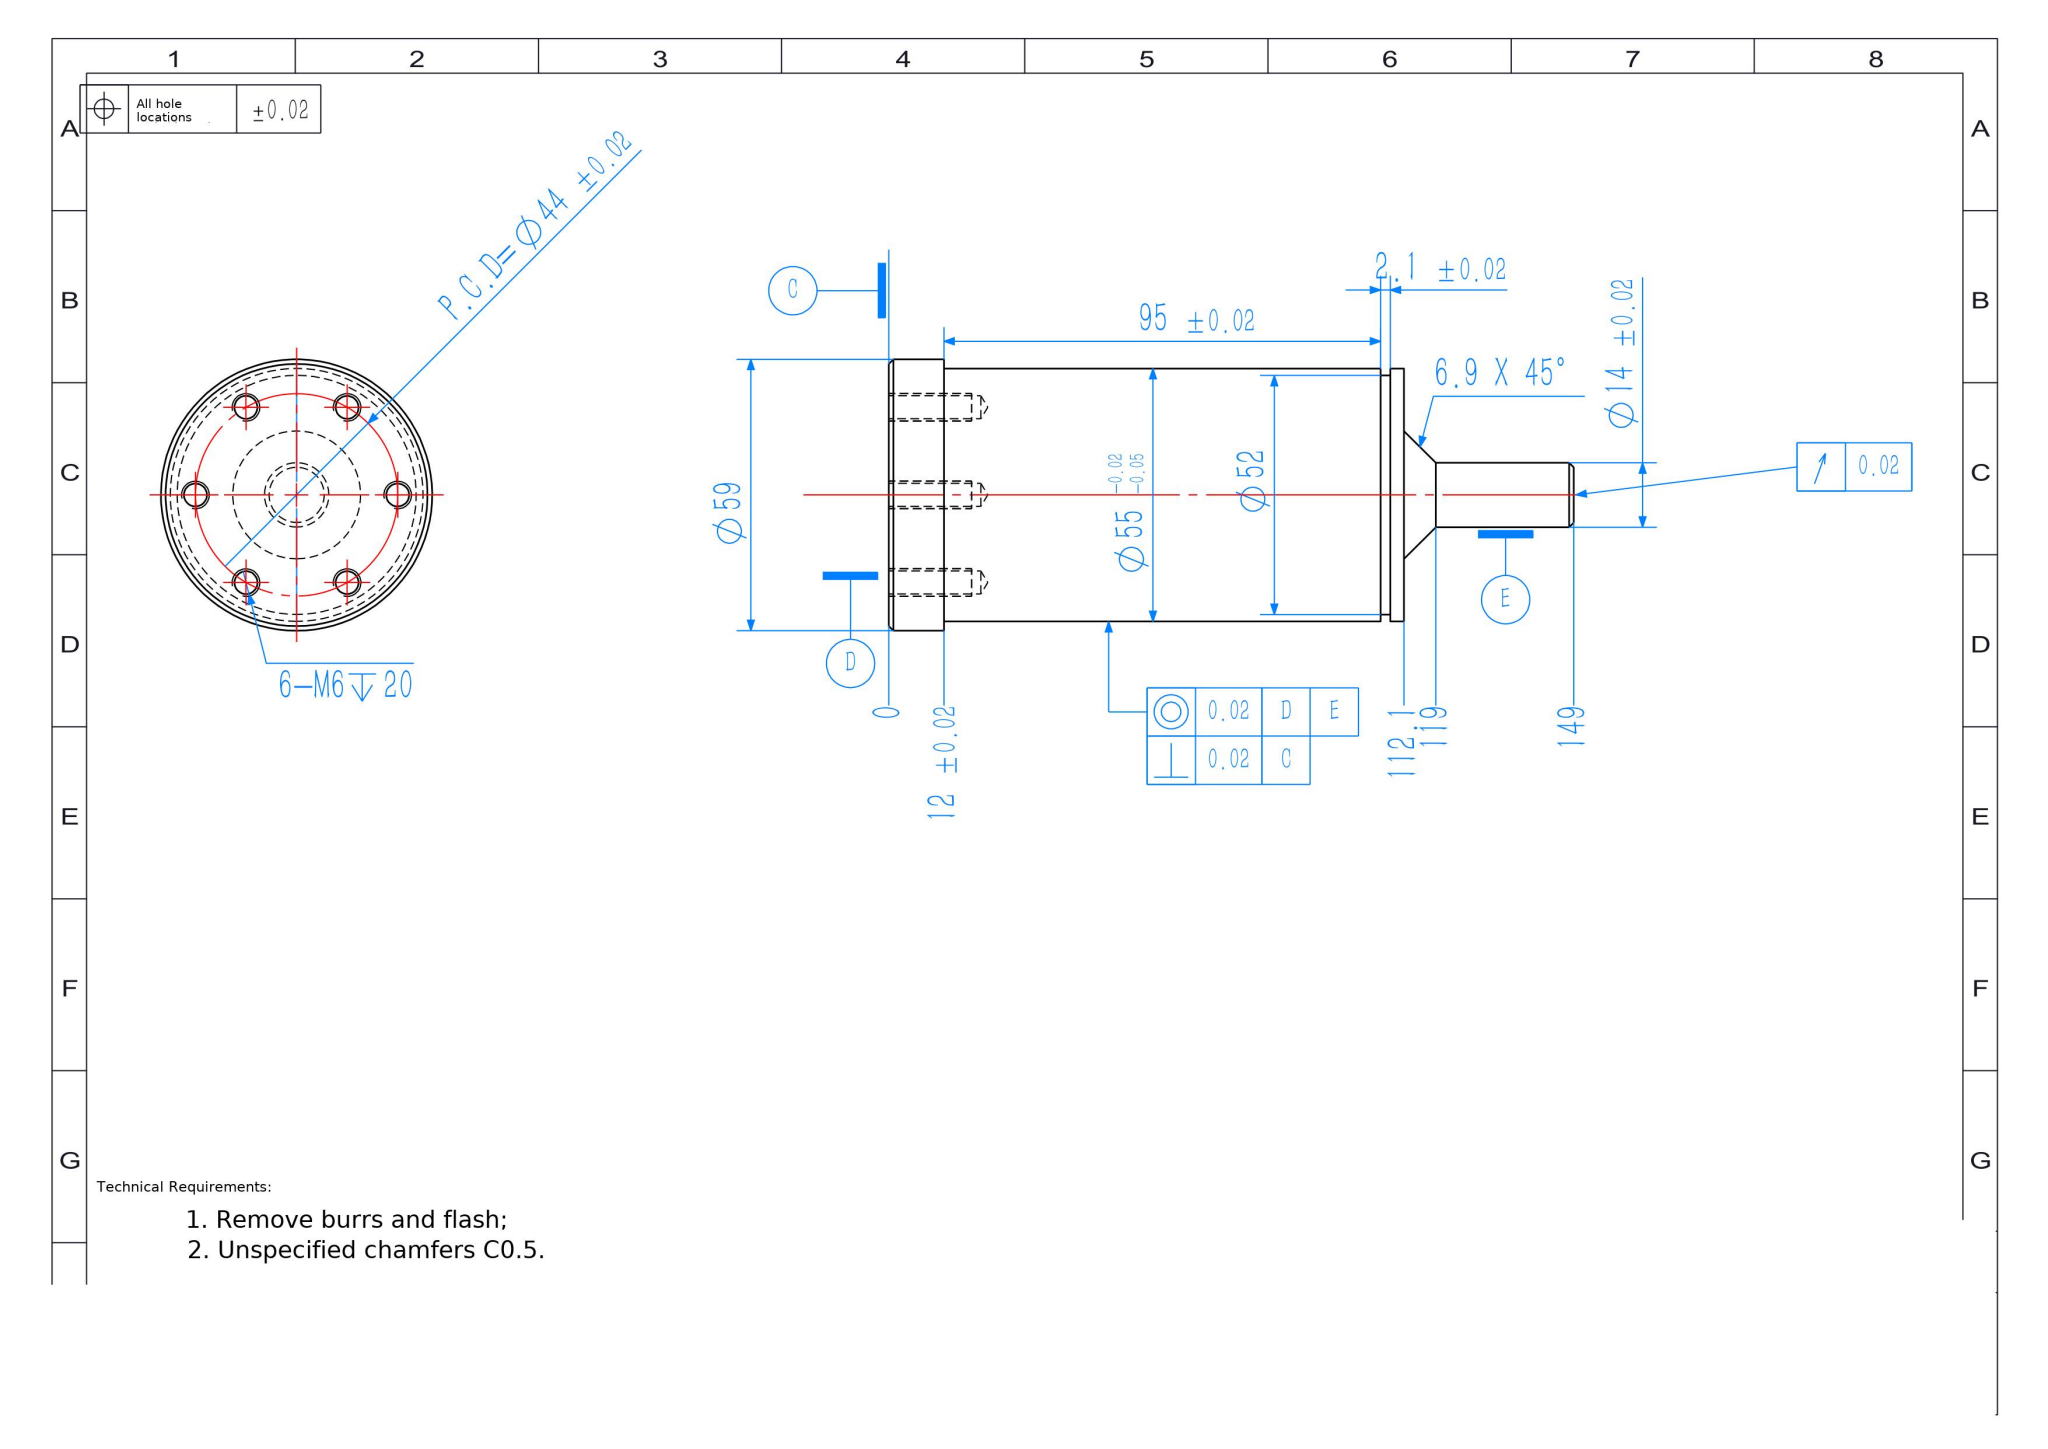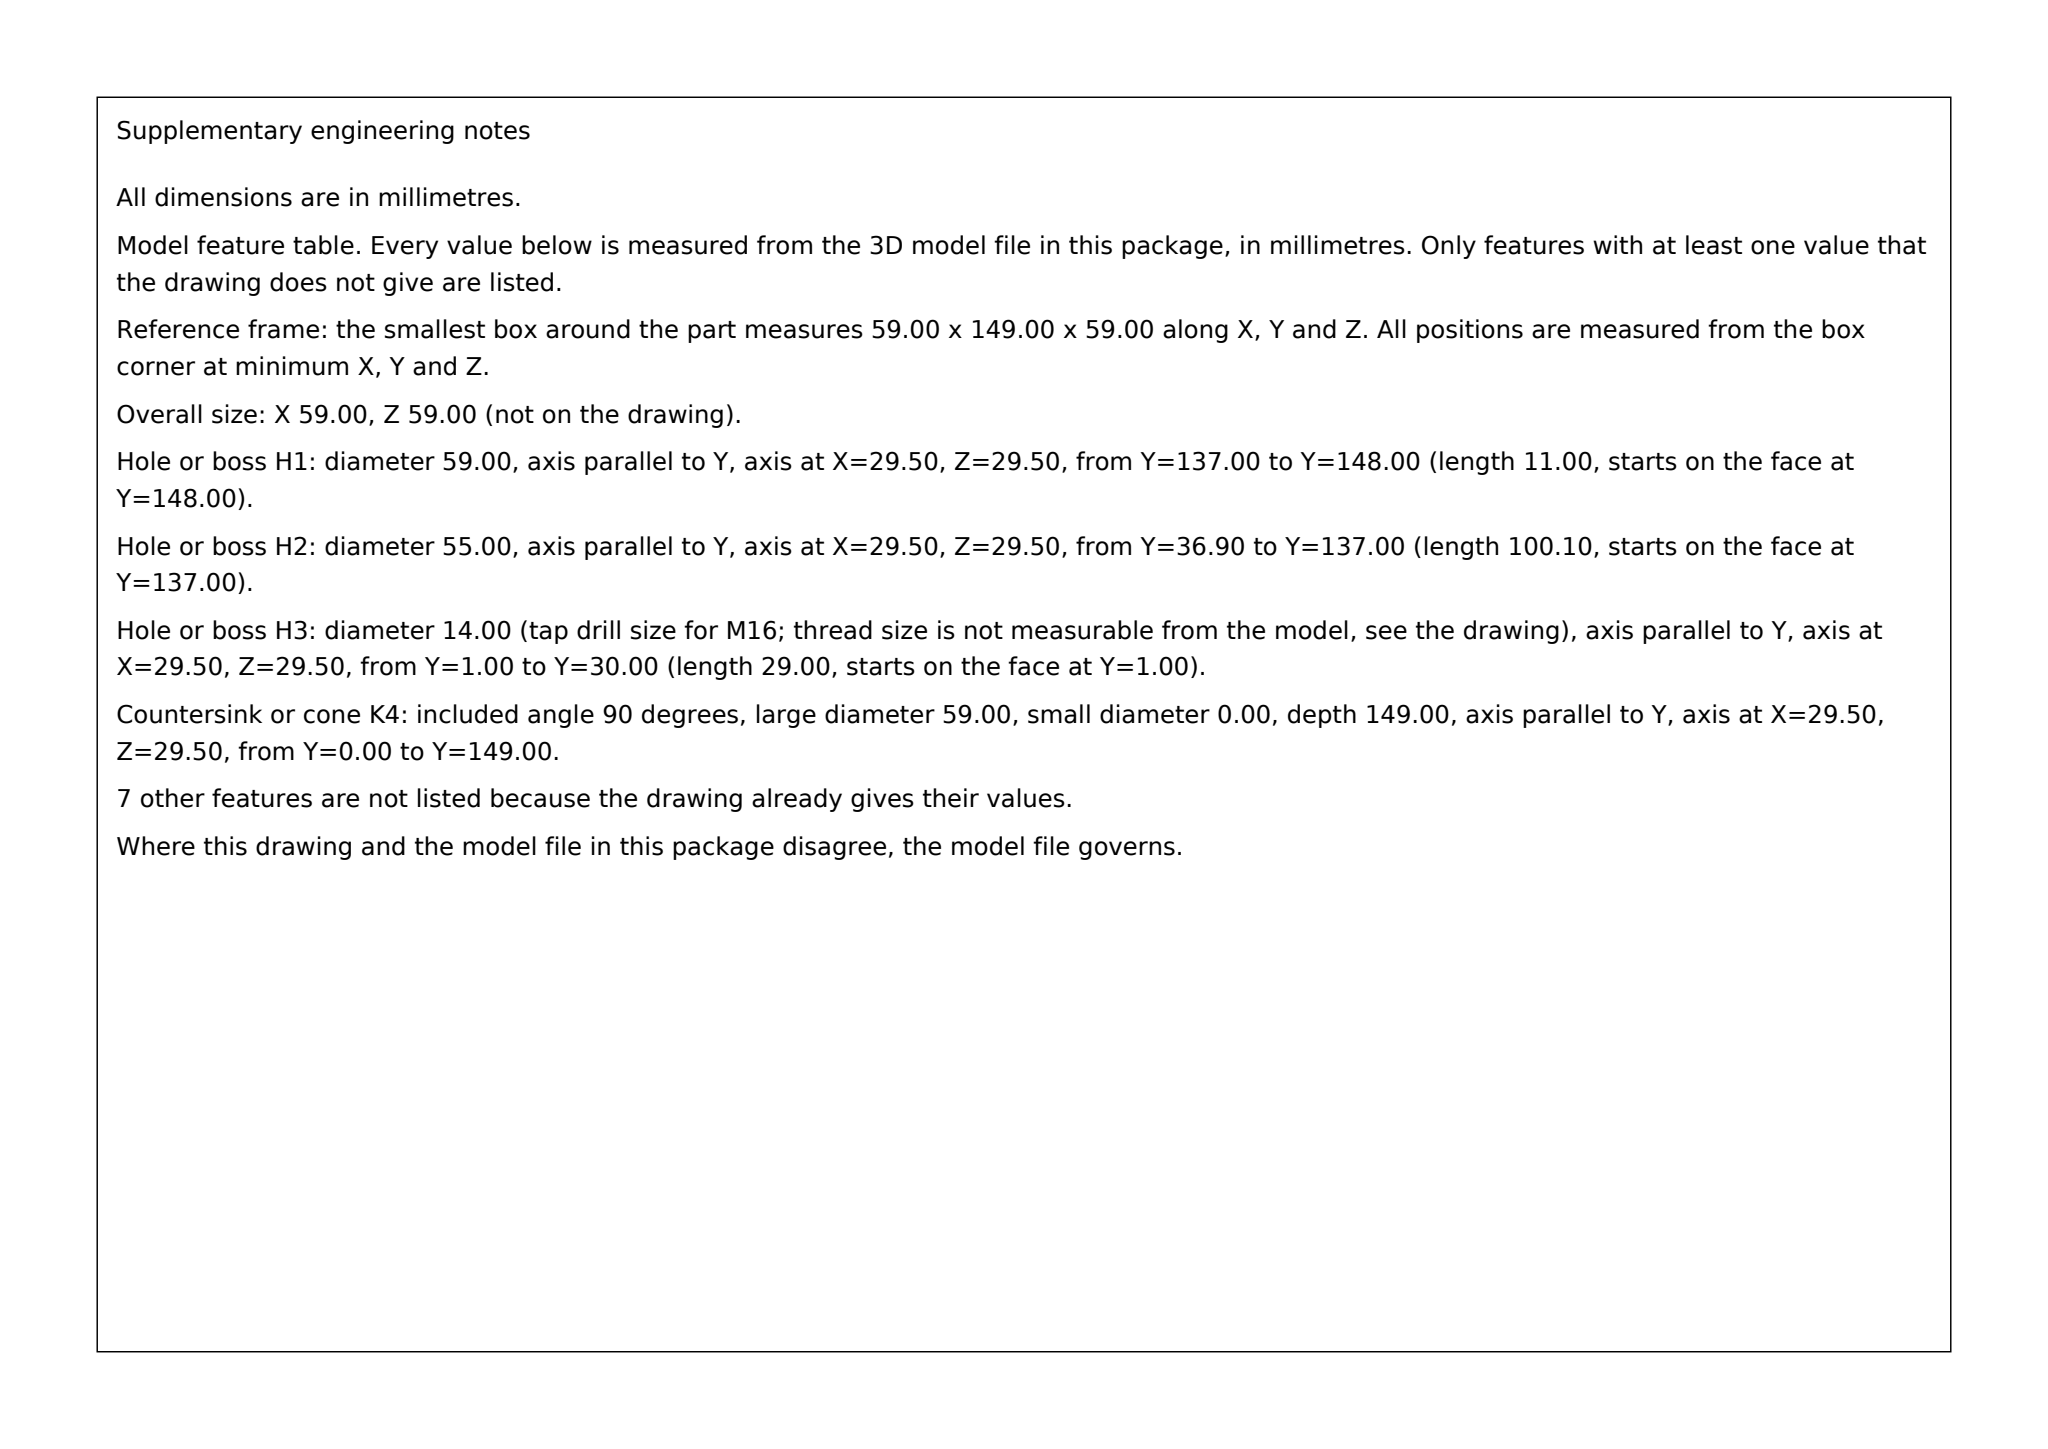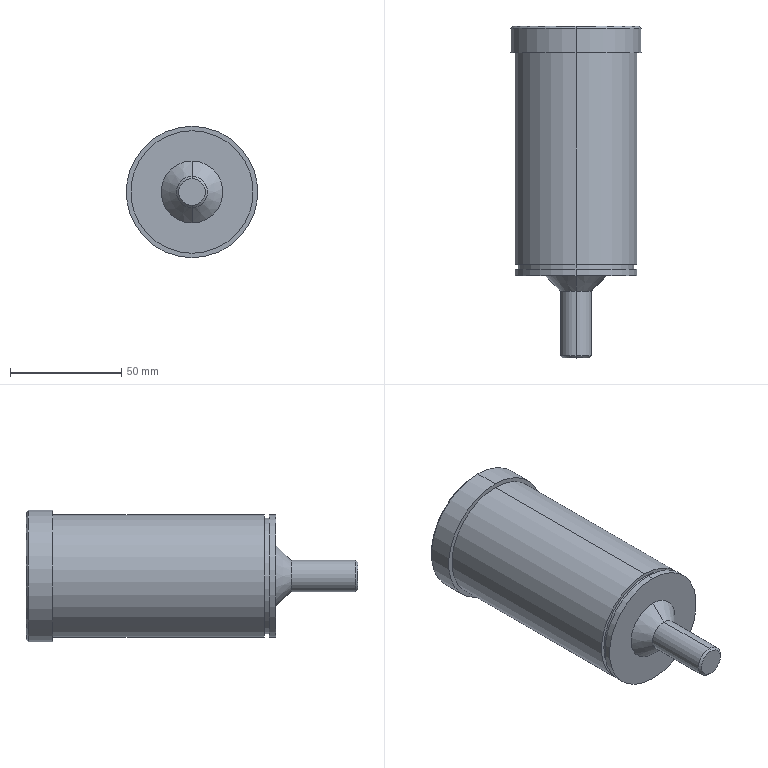Part | SolidWorks | mm | 1 solid | 46 faces | box 59 x 149 x 59 mm | volume 274642 mm3 | cylinder 22 | cone 18 | plane 6 | commonest cylinder face diameters 5 x12 55 x4 14 x2 52 x2 59 x2
build123d program:
from build123d import *

# Parameters (mm, degrees)
SKETCH1_R           = 29.5
BOSS_EXTRUDE1_DEPTH = 149
SKETCH2_W           = 2
SKETCH2_H           = 137
SKETCH3_W           = 1.5
SKETCH3_H           = 2.1
CIRPATTERN1_COUNT   = 6
CHAMFER2_SIZE       = 1


with BuildPart() as part:
    # Sketch1 → Boss-Extrude1 (new body)
    with BuildSketch(Plane(origin=(0, 0, 0), x_dir=(1, 0, 0), z_dir=(0, 1, 0))):
        with Locations(Location((0, 0, 0), (0, 0, 270))):
            Circle(SKETCH1_R)
    extrude(amount=BOSS_EXTRUDE1_DEPTH)

    # Sketch2 → Cut-Revolve1 (revolve, cut)
    with BuildSketch(Plane.XY, mode=Mode.PRIVATE) as cut_revolve1_sk:
        with Locations((28.5, 68.5)):
            Rectangle(SKETCH2_W, SKETCH2_H)
    revolve(cut_revolve1_sk.sketch.rotate(Axis((0, 149, 0), (0, -1, 0)), 90), axis=Axis((0, 149, 0), (0, -1, 0)), mode=Mode.SUBTRACT)

    # Sketch3 → Cut-Revolve2 (revolve, cut)
    with BuildSketch(Plane.XY, mode=Mode.PRIVATE) as cut_revolve2_sk:
        with Locations((26.75, 40.95)):
            Rectangle(SKETCH3_W, SKETCH3_H)
        Polygon((7, 0), (7, 30), (13.9, 36.9), (27.5, 36.9), (27.5, 0), align=None)
    revolve(cut_revolve2_sk.sketch.rotate(Axis((0, 149, 0), (0, -1, 0)), 90), axis=Axis((0, 149, 0), (0, -1, 0)), mode=Mode.SUBTRACT)

    # Sketch5 → M6 Tapped Hole1 (revolve, cut)
    with BuildSketch(Plane(origin=(-11, 149, -19.053), x_dir=(0, 0, 1), z_dir=(1, 0, 0))):
        Polygon((0, 0), (0, 21.502), (2.5, 20), (2.5, 0), align=None)
    m6_tapped_hole1 = revolve(axis=Axis((-11, 155.35, -19.053), (0, -1, 0)), mode=Mode.SUBTRACT)

    # CirPattern1: M6 Tapped Hole1 ×6 about axis
    cirpattern1_axis = Axis((0, 0, 0), (0, 1, 0))
    for i in range(1, CIRPATTERN1_COUNT):
        add(m6_tapped_hole1.rotate(cirpattern1_axis, i * 360 / CIRPATTERN1_COUNT), mode=Mode.SUBTRACT)

    # Chamfer2
    chamfer2_edges = [part.edges().sort_by_distance(p)[0] for p in [
        (0, 0, -7),
        (0, 149, -29.5),
    ]]
    chamfer(chamfer2_edges, length=CHAMFER2_SIZE)


solid = part.part